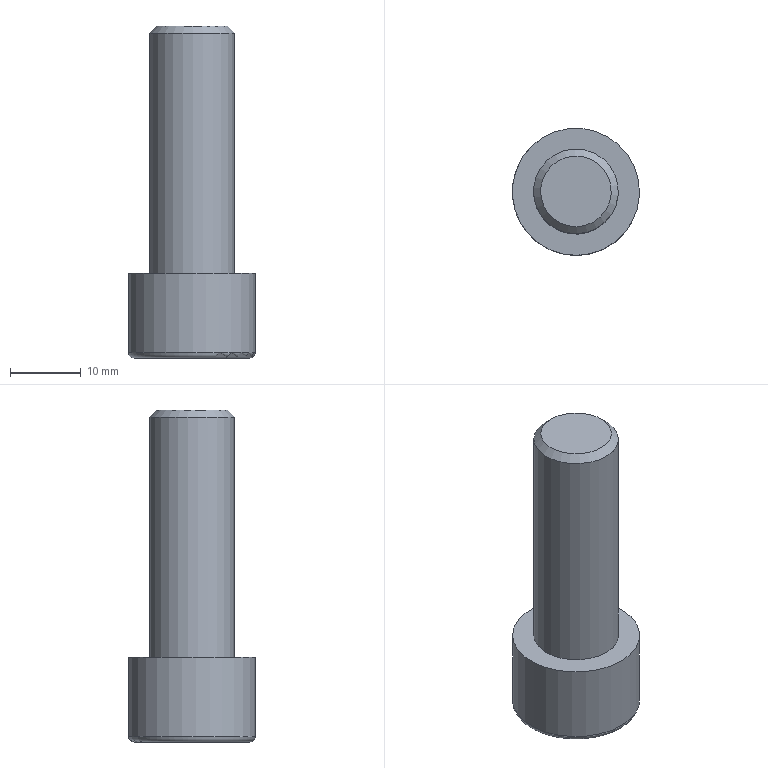Component | NX | GB_T70_1_M12X35 | 1 solid | 20 faces | volume 6253 mm3 | plane 15 | cylinder 2 | cone 2 | torus 1 | commonest cylinder face diameters 18 x1 12 x1